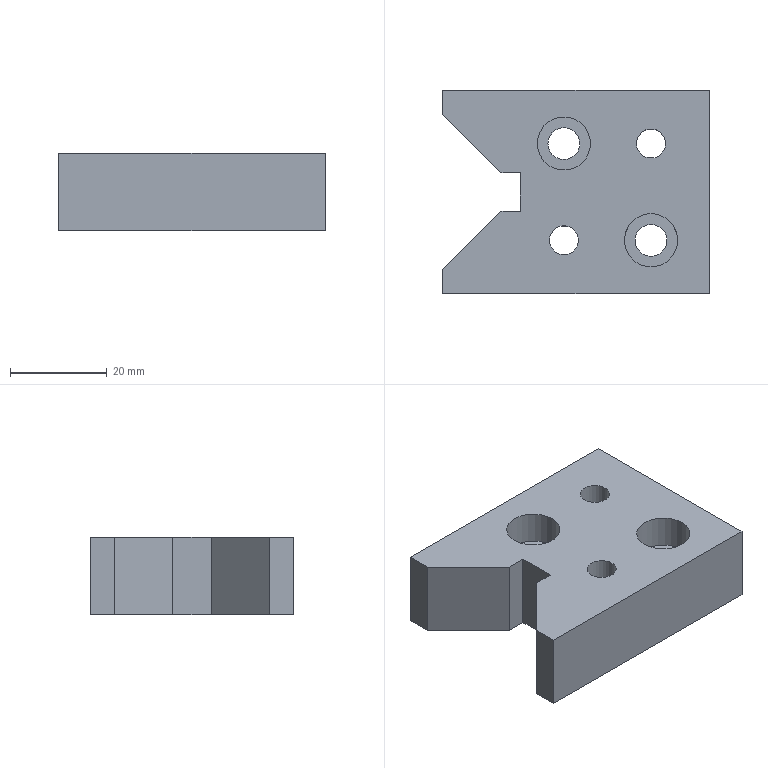Component | NX | FIXED_V_BLOCK | 1 solid | 20 faces | volume 29781 mm3 | plane 14 | cylinder 6 | commonest cylinder face diameters 6.6 x2 11 x2 6 x2